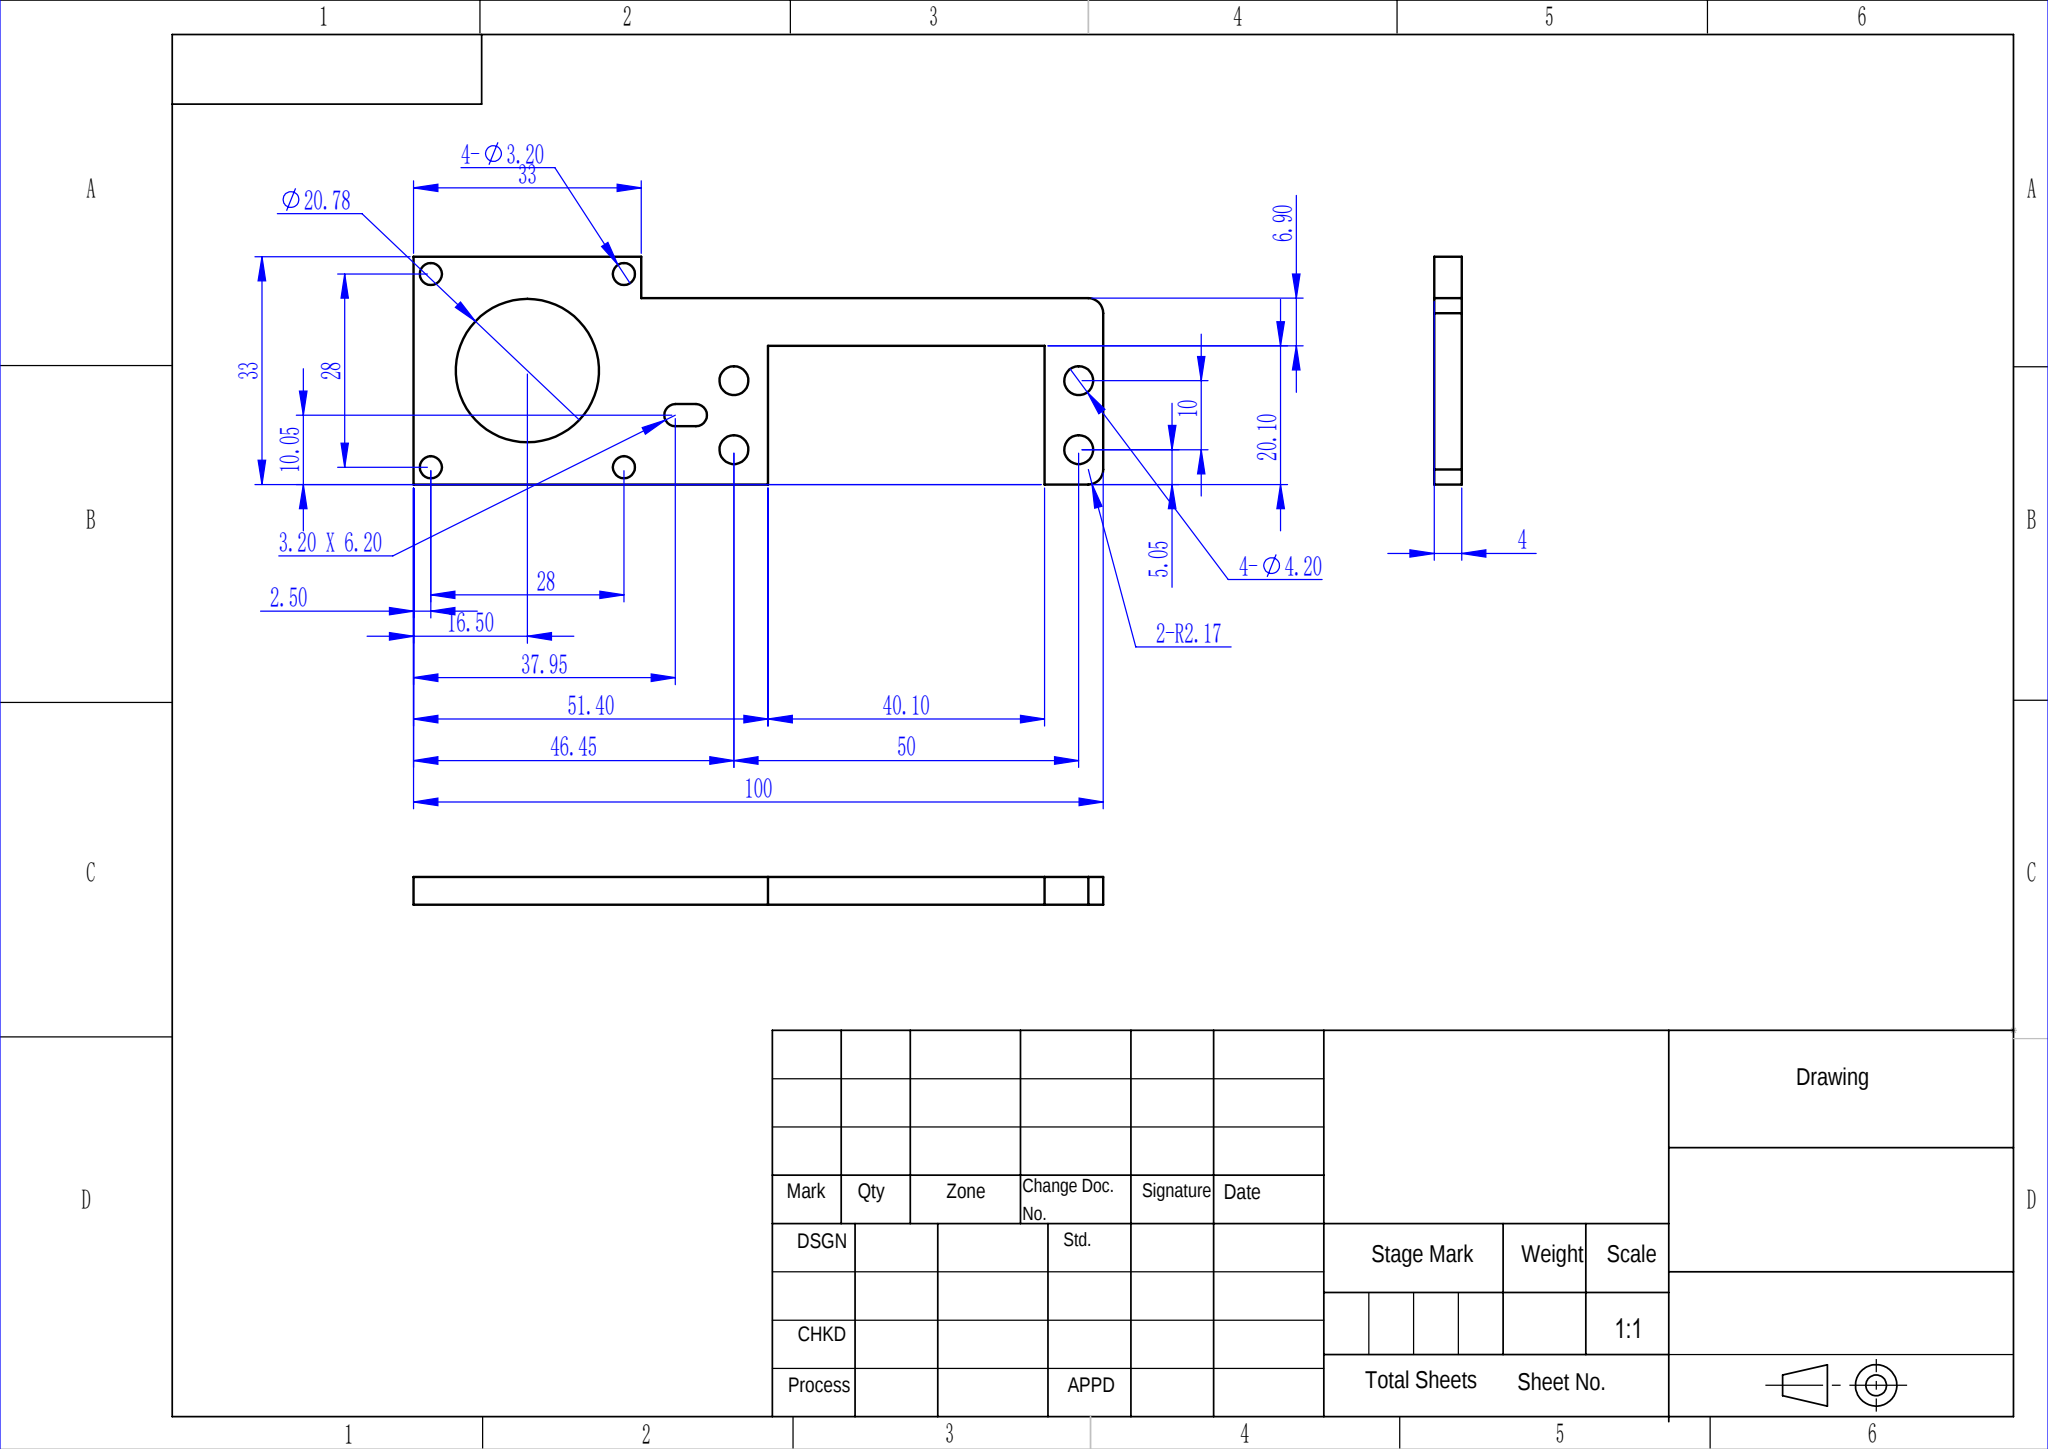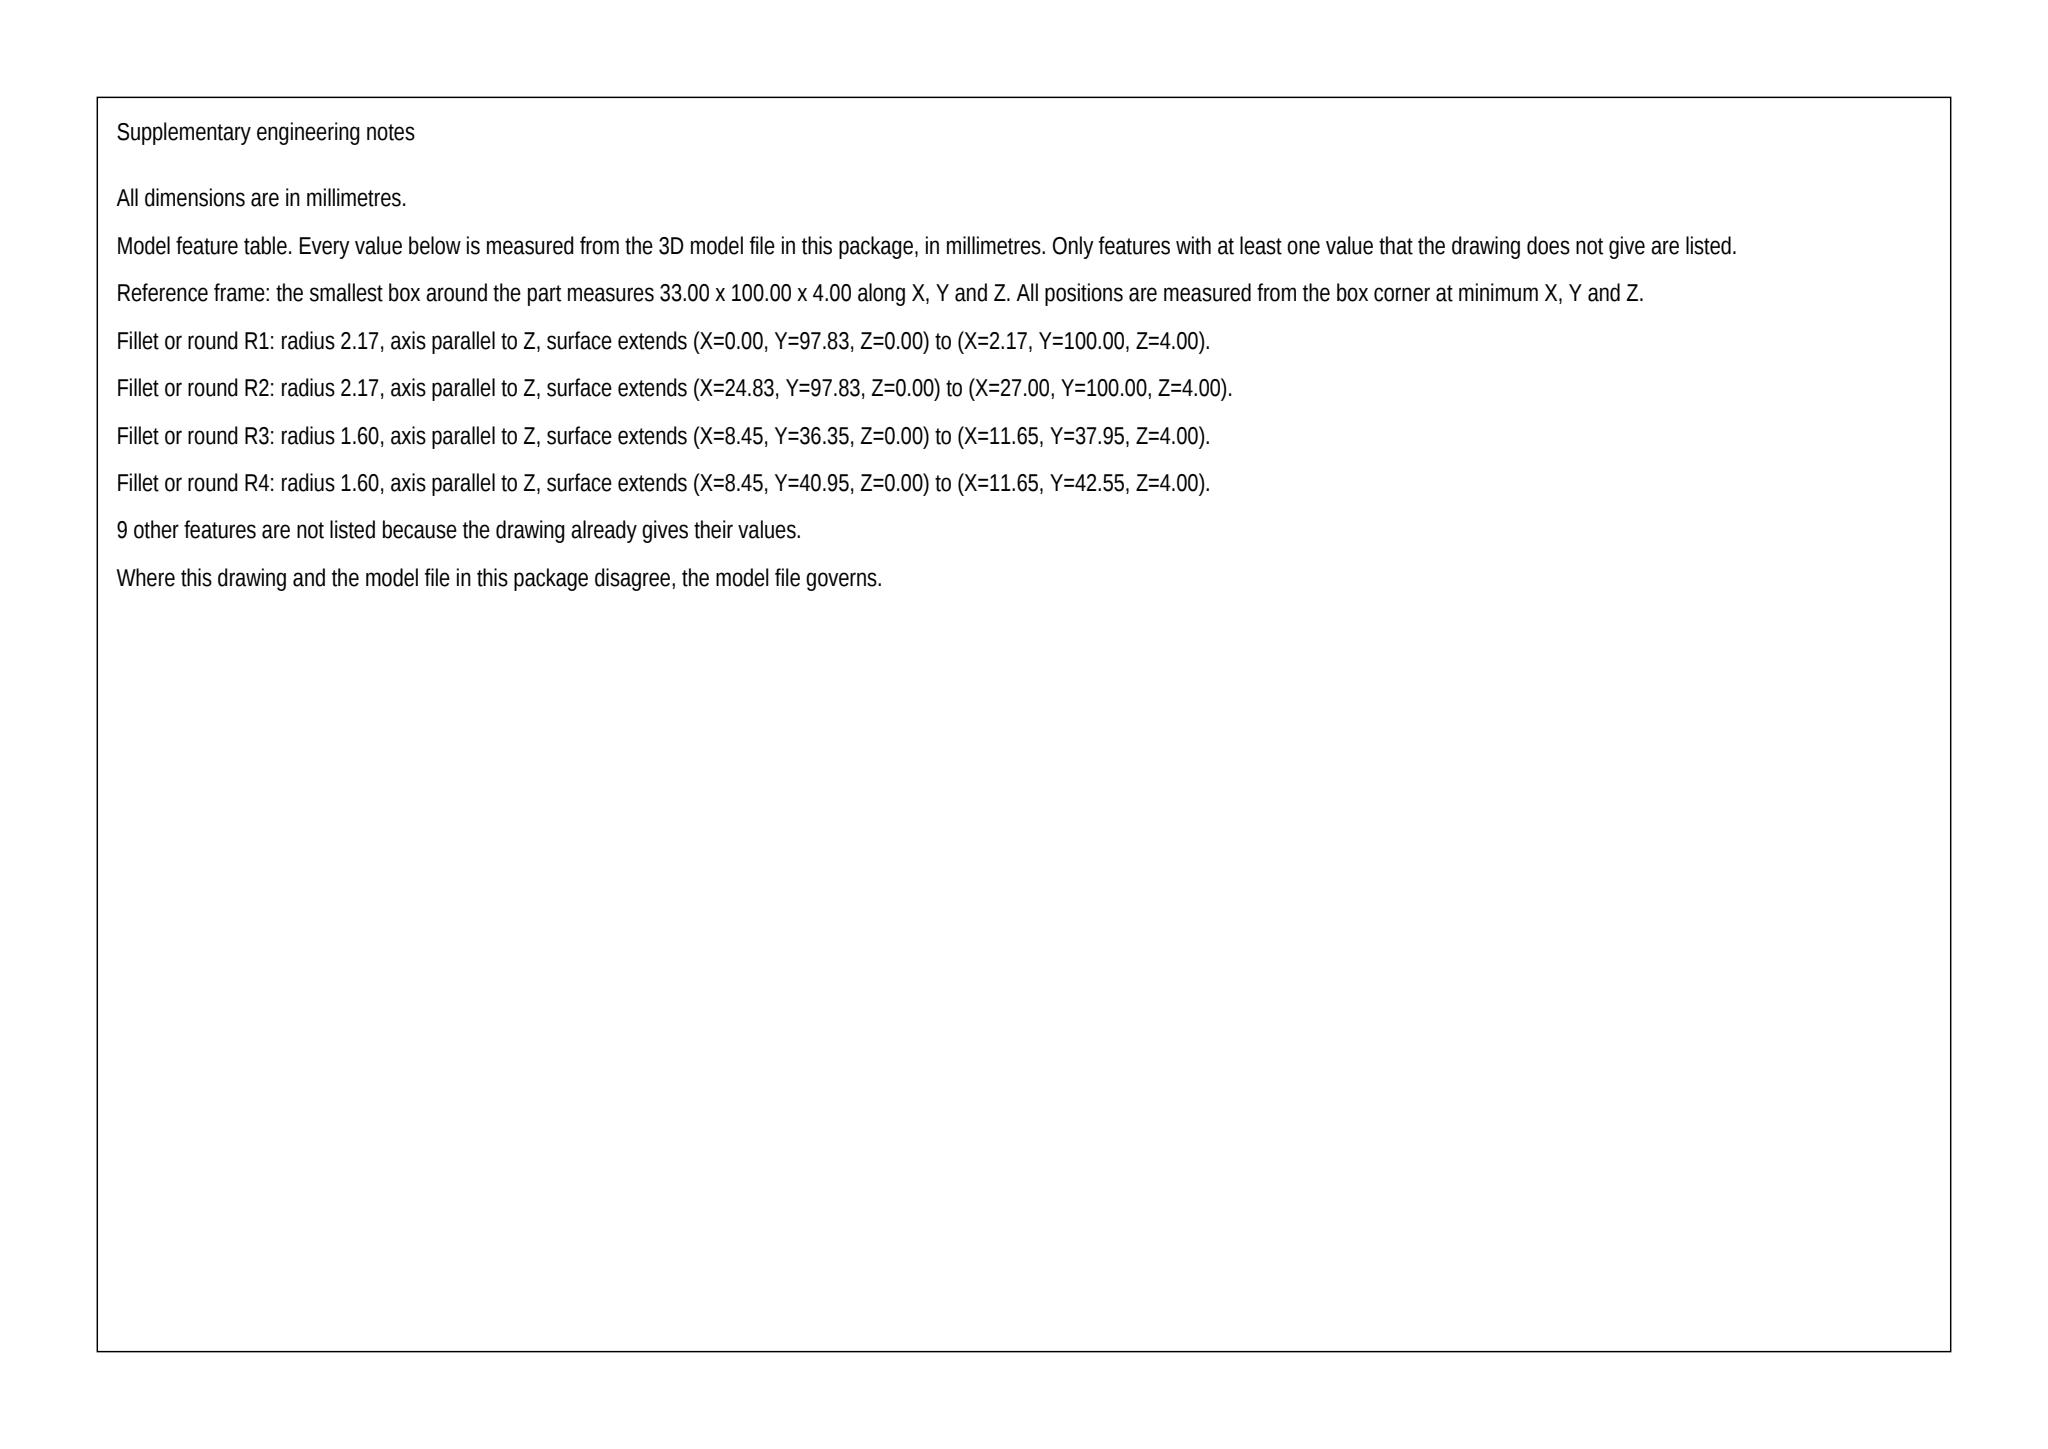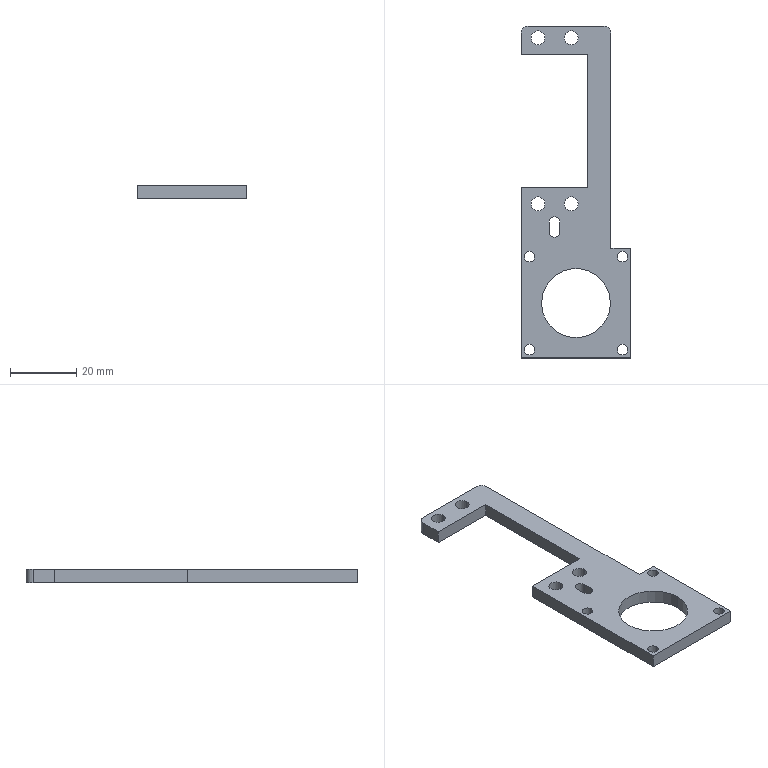Part | SolidWorks | mm | 1 solid | 36 faces | box 33 x 100 x 4 mm | volume 6582 mm3 | cylinder 22 | plane 14 | commonest cylinder face diameters 3.2 x10 4.2 x8 20.781 x2 4.332 x2
build123d program:
from build123d import *

# Parameters (mm, degrees)
SKETCH1_R           = 2.1
SKETCH1_R_2         = 1.6
SKETCH1_R_3         = 10.39
BOSS_EXTRUDE1_DEPTH = 4


with BuildPart() as part:
    # Sketch1 → Boss-Extrude1 (new body)
    with BuildSketch(Plane.XY):
        with BuildLine():
            Line((-5.552, -19.876), (-5.552, -34.206))
            Line((-5.552, -34.206), (-5.552, -71.276))
            Line((-5.552, -71.276), (21.448, -71.276))
            Line((21.448, -71.276), (27.448, -71.276))
            Line((27.448, -71.276), (27.448, -38.276))
            Line((27.448, -38.276), (21.448, -38.276))
            Line((21.448, -38.276), (21.448, 26.558))
            ThreePointArc((21.448, 26.558), (20.814, 28.09), (19.282, 28.724))
            Line((19.282, 28.724), (-3.386, 28.724))
            ThreePointArc((-3.386, 28.724), (-4.918, 28.09), (-5.552, 26.558))
            Line((-5.552, 26.558), (-5.552, 20.224))
            Line((-5.552, 20.224), (14.548, 20.224))
            Line((14.548, 20.224), (14.548, -19.876))
            Line((14.548, -19.876), (-5.552, -19.876))
        make_face()
        with Locations((-0.502, 25.174)):
            Circle(SKETCH1_R, mode=Mode.SUBTRACT)
        with Locations((9.498, 25.174)):
            Circle(SKETCH1_R, mode=Mode.SUBTRACT)
        with Locations((-0.502, -24.826)):
            Circle(SKETCH1_R, mode=Mode.SUBTRACT)
        with Locations((9.498, -24.826)):
            Circle(SKETCH1_R, mode=Mode.SUBTRACT)
        with Locations((-3.052, -40.776)):
            Circle(SKETCH1_R_2, mode=Mode.SUBTRACT)
        with Locations((24.948, -40.776)):
            Circle(SKETCH1_R_2, mode=Mode.SUBTRACT)
        with Locations((-3.052, -68.776)):
            Circle(SKETCH1_R_2, mode=Mode.SUBTRACT)
        with Locations((24.948, -68.776)):
            Circle(SKETCH1_R_2, mode=Mode.SUBTRACT)
        with Locations((10.948, -54.776)):
            Circle(SKETCH1_R_3, mode=Mode.SUBTRACT)
        with BuildLine():
            Line((6.098, -30.326), (6.098, -33.326))
            ThreePointArc((6.098, -33.326), (4.498, -34.926), (2.898, -33.326))
            Line((2.898, -33.326), (2.898, -30.326))
            ThreePointArc((2.898, -30.326), (4.498, -28.726), (6.098, -30.326))
        make_face(mode=Mode.SUBTRACT)
    extrude(amount=BOSS_EXTRUDE1_DEPTH)


solid = part.part